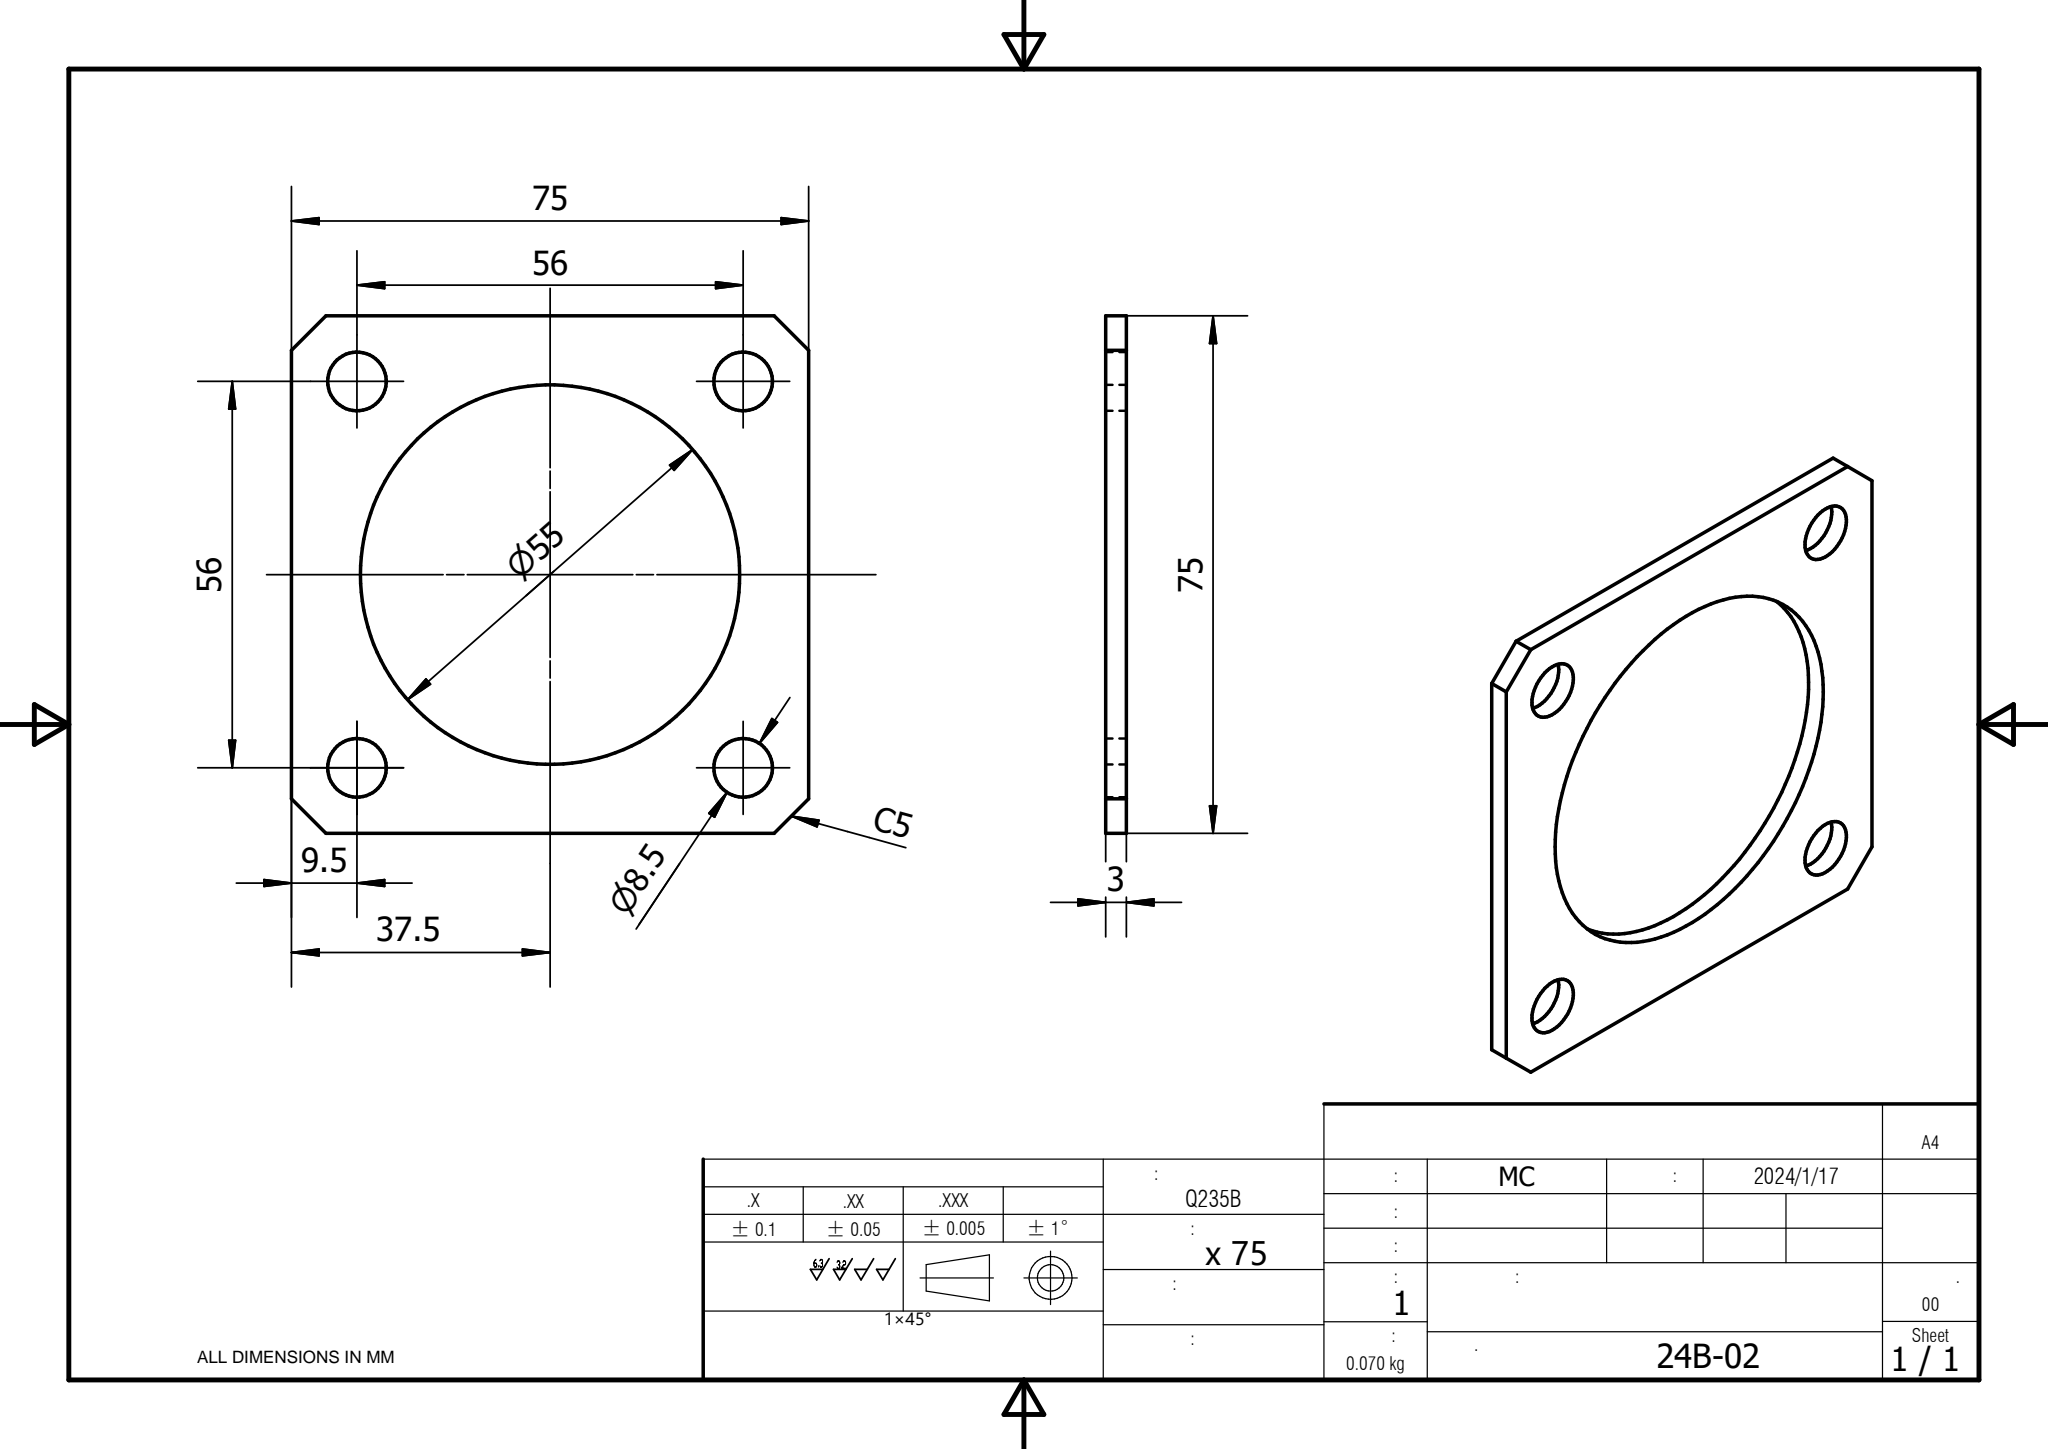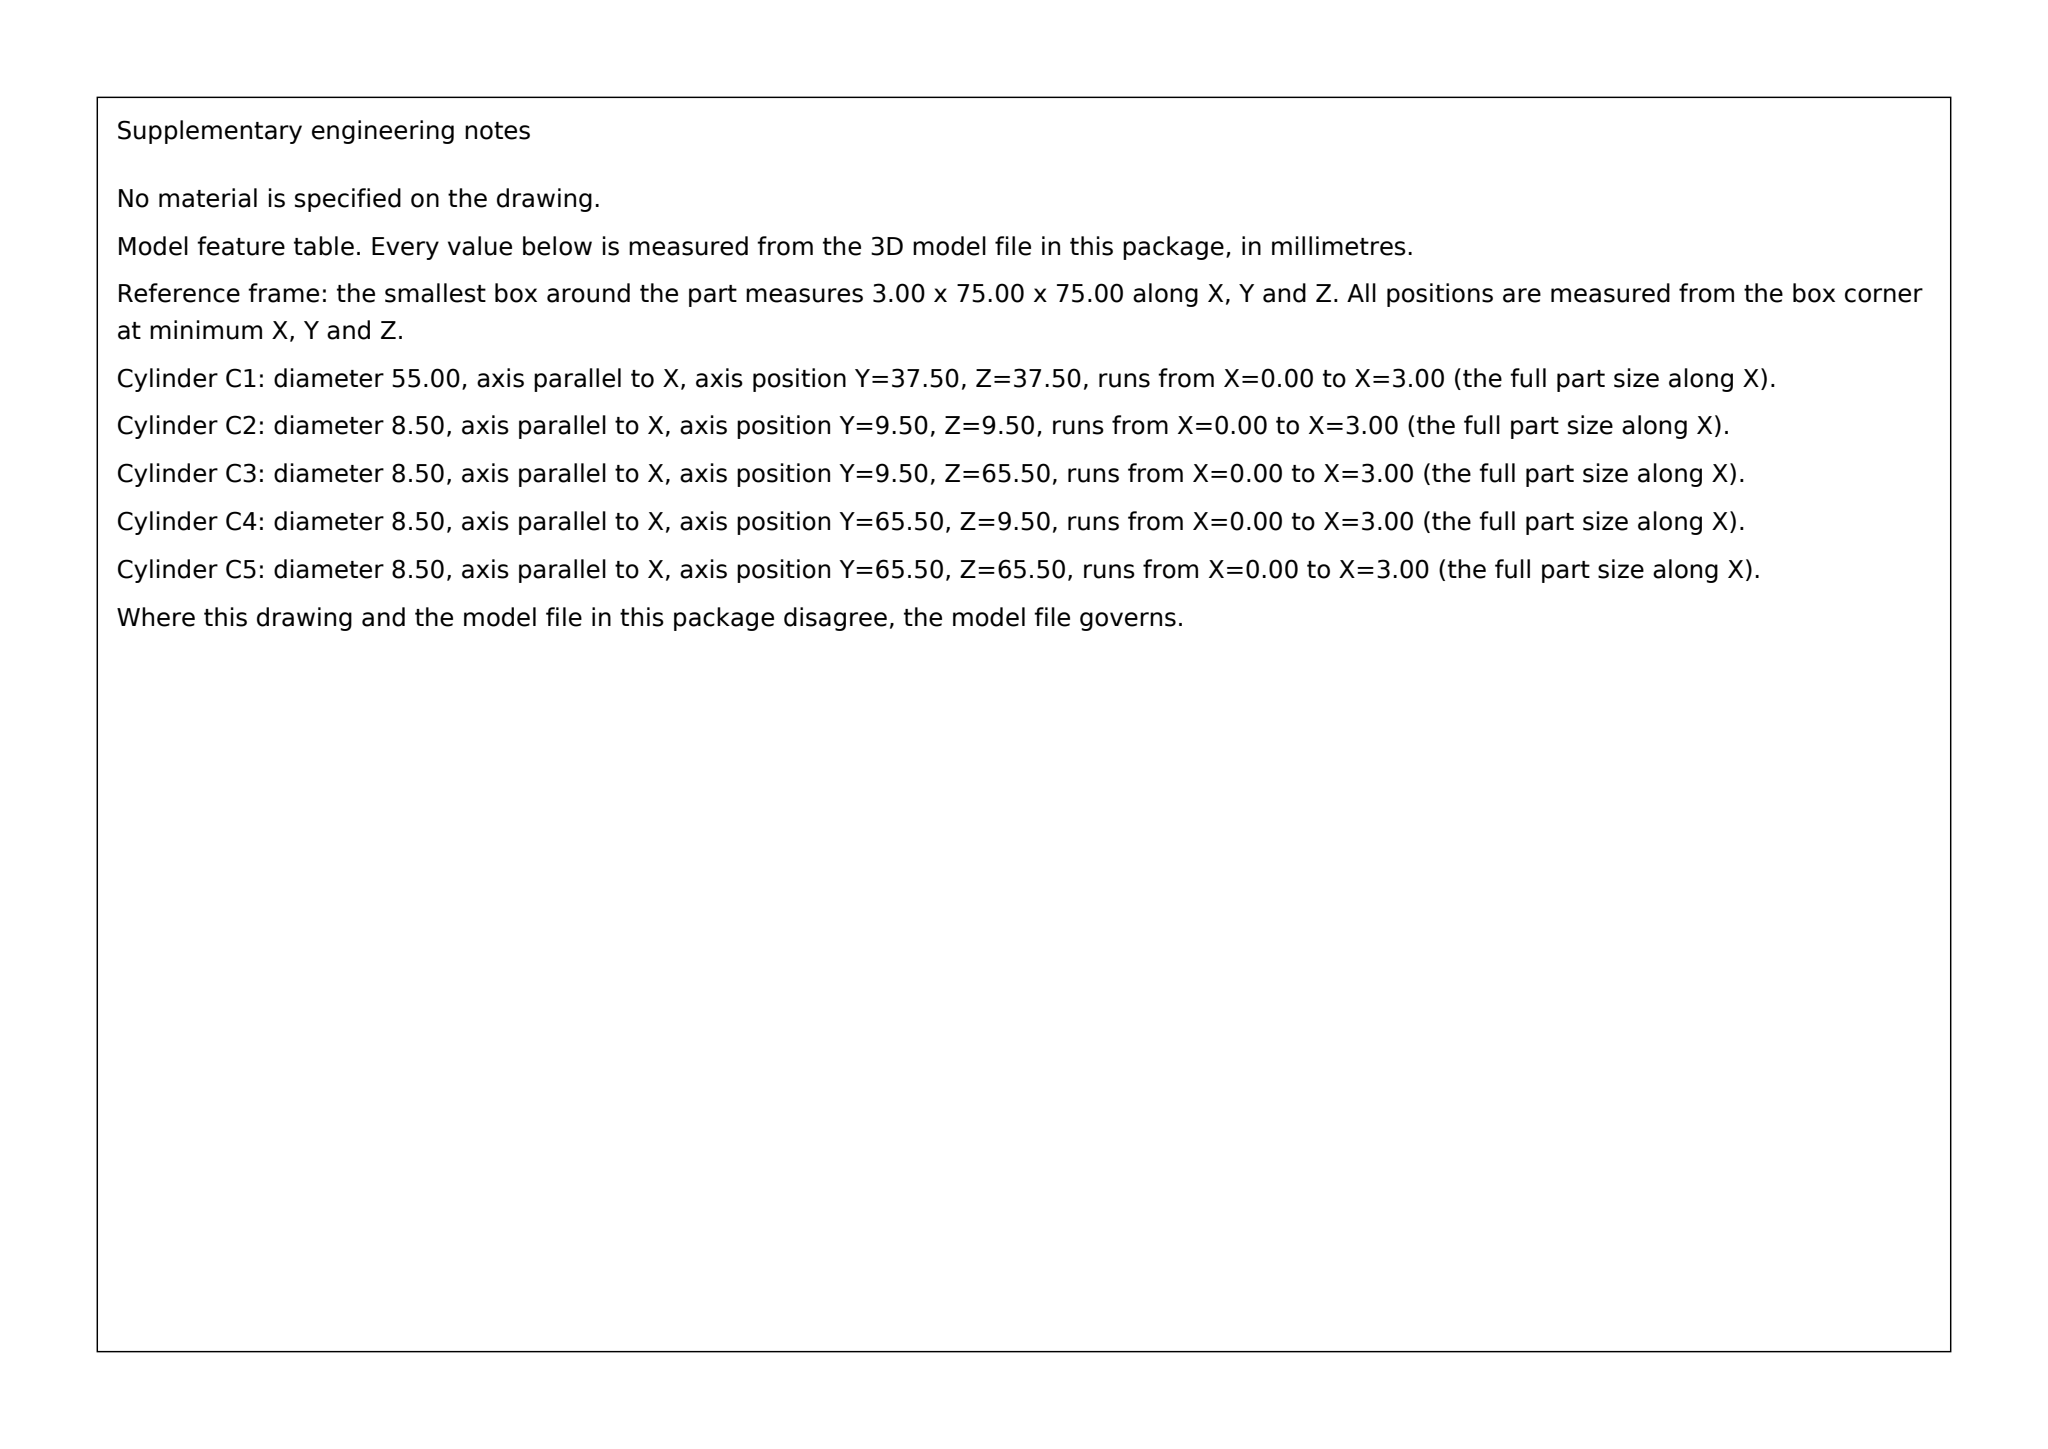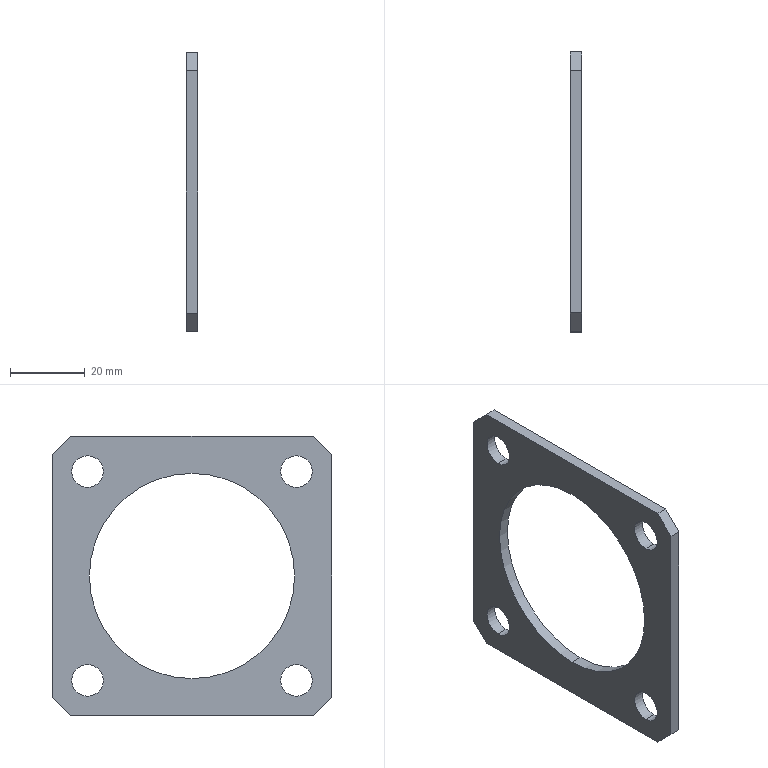Part | SolidWorks | mm | material Q235B | 1 solid | 20 faces | box 3 x 75 x 75 mm | volume 8917 mm3 | cylinder 10 | plane 10 | commonest cylinder face diameters 8.5 x8 55 x2
STEP:
#1=CARTESIAN_POINT('',(3.,0.,-27.5));
#2=VERTEX_POINT('',#1);
#3=CARTESIAN_POINT('',(3.,0.,27.5));
#4=VERTEX_POINT('',#3);
#5=CARTESIAN_POINT('',(3.,0.,0.));
#6=DIRECTION('',(-1.,0.,0.));
#7=DIRECTION('',(0.,0.,1.));
#8=AXIS2_PLACEMENT_3D('',#5,#6,#7);
#9=CIRCLE('',#8,27.5);
#10=EDGE_CURVE('',#2,#4,#9,.T.);
#11=ORIENTED_EDGE('',*,*,#10,.F.);
#12=CARTESIAN_POINT('',(0.,0.,-27.5));
#13=VERTEX_POINT('',#12);
#14=CARTESIAN_POINT('',(3.,0.,-27.5));
#15=DIRECTION('',(-1.,0.,0.));
#16=VECTOR('',#15,1000.);
#17=LINE('',#14,#16);
#18=EDGE_CURVE('',#2,#13,#17,.T.);
#19=ORIENTED_EDGE('',*,*,#18,.T.);
#20=CARTESIAN_POINT('',(0.,0.,27.5));
#21=VERTEX_POINT('',#20);
#22=CARTESIAN_POINT('',(0.,0.,0.));
#23=DIRECTION('',(-1.,0.,0.));
#24=DIRECTION('',(0.,0.,1.));
#25=AXIS2_PLACEMENT_3D('',#22,#23,#24);
#26=CIRCLE('',#25,27.5);
#27=EDGE_CURVE('',#13,#21,#26,.T.);
#28=ORIENTED_EDGE('',*,*,#27,.T.);
#29=CARTESIAN_POINT('',(3.,0.,27.5));
#30=DIRECTION('',(-1.,0.,0.));
#31=VECTOR('',#30,1000.);
#32=LINE('',#29,#31);
#33=EDGE_CURVE('',#4,#21,#32,.T.);
#34=ORIENTED_EDGE('',*,*,#33,.F.);
#35=EDGE_LOOP('',(#11,#19,#28,#34));
#36=FACE_OUTER_BOUND('',#35,.T.);
#37=CARTESIAN_POINT('',(3.,0.,0.));
#38=DIRECTION('',(-1.,0.,0.));
#39=DIRECTION('',(0.,0.,1.));
#40=AXIS2_PLACEMENT_3D('',#37,#38,#39);
#41=CYLINDRICAL_SURFACE('',#40,27.5);
#42=ADVANCED_FACE('',(#36),#41,.F.);
#43=CARTESIAN_POINT('',(0.,-28.,-32.25));
#44=VERTEX_POINT('',#43);
#45=CARTESIAN_POINT('',(0.,-28.,-23.75));
#46=VERTEX_POINT('',#45);
#47=CARTESIAN_POINT('',(0.,-28.,-28.));
#48=DIRECTION('',(-1.,0.,0.));
#49=DIRECTION('',(0.,0.,-1.));
#50=AXIS2_PLACEMENT_3D('',#47,#48,#49);
#51=CIRCLE('',#50,4.25);
#52=EDGE_CURVE('',#44,#46,#51,.T.);
#53=ORIENTED_EDGE('',*,*,#52,.T.);
#54=CARTESIAN_POINT('',(3.,-28.,-23.75));
#55=VERTEX_POINT('',#54);
#56=CARTESIAN_POINT('',(-103.108,-28.,-23.75));
#57=DIRECTION('',(1.,0.,0.));
#58=VECTOR('',#57,1000.);
#59=LINE('',#56,#58);
#60=EDGE_CURVE('',#46,#55,#59,.T.);
#61=ORIENTED_EDGE('',*,*,#60,.T.);
#62=CARTESIAN_POINT('',(3.,-28.,-32.25));
#63=VERTEX_POINT('',#62);
#64=CARTESIAN_POINT('',(3.,-28.,-28.));
#65=DIRECTION('',(-1.,0.,0.));
#66=DIRECTION('',(0.,0.,-1.));
#67=AXIS2_PLACEMENT_3D('',#64,#65,#66);
#68=CIRCLE('',#67,4.25);
#69=EDGE_CURVE('',#63,#55,#68,.T.);
#70=ORIENTED_EDGE('',*,*,#69,.F.);
#71=CARTESIAN_POINT('',(-103.108,-28.,-32.25));
#72=DIRECTION('',(1.,0.,0.));
#73=VECTOR('',#72,1000.);
#74=LINE('',#71,#73);
#75=EDGE_CURVE('',#44,#63,#74,.T.);
#76=ORIENTED_EDGE('',*,*,#75,.F.);
#77=EDGE_LOOP('',(#53,#61,#70,#76));
#78=FACE_OUTER_BOUND('',#77,.T.);
#79=CARTESIAN_POINT('',(-103.108,-28.,-28.));
#80=DIRECTION('',(1.,0.,0.));
#81=DIRECTION('',(0.,0.,-1.));
#82=AXIS2_PLACEMENT_3D('',#79,#80,#81);
#83=CYLINDRICAL_SURFACE('',#82,4.25);
#84=ADVANCED_FACE('',(#78),#83,.F.);
#85=CARTESIAN_POINT('',(0.,28.,-32.25));
#86=VERTEX_POINT('',#85);
#87=CARTESIAN_POINT('',(0.,28.,-23.75));
#88=VERTEX_POINT('',#87);
#89=CARTESIAN_POINT('',(0.,28.,-28.));
#90=DIRECTION('',(-1.,0.,0.));
#91=DIRECTION('',(0.,0.,-1.));
#92=AXIS2_PLACEMENT_3D('',#89,#90,#91);
#93=CIRCLE('',#92,4.25);
#94=EDGE_CURVE('',#86,#88,#93,.T.);
#95=ORIENTED_EDGE('',*,*,#94,.T.);
#96=CARTESIAN_POINT('',(3.,28.,-23.75));
#97=VERTEX_POINT('',#96);
#98=CARTESIAN_POINT('',(-103.108,28.,-23.75));
#99=DIRECTION('',(1.,0.,0.));
#100=VECTOR('',#99,1000.);
#101=LINE('',#98,#100);
#102=EDGE_CURVE('',#88,#97,#101,.T.);
#103=ORIENTED_EDGE('',*,*,#102,.T.);
#104=CARTESIAN_POINT('',(3.,28.,-32.25));
#105=VERTEX_POINT('',#104);
#106=CARTESIAN_POINT('',(3.,28.,-28.));
#107=DIRECTION('',(-1.,0.,0.));
#108=DIRECTION('',(0.,0.,-1.));
#109=AXIS2_PLACEMENT_3D('',#106,#107,#108);
#110=CIRCLE('',#109,4.25);
#111=EDGE_CURVE('',#105,#97,#110,.T.);
#112=ORIENTED_EDGE('',*,*,#111,.F.);
#113=CARTESIAN_POINT('',(-103.108,28.,-32.25));
#114=DIRECTION('',(1.,0.,0.));
#115=VECTOR('',#114,1000.);
#116=LINE('',#113,#115);
#117=EDGE_CURVE('',#86,#105,#116,.T.);
#118=ORIENTED_EDGE('',*,*,#117,.F.);
#119=EDGE_LOOP('',(#95,#103,#112,#118));
#120=FACE_OUTER_BOUND('',#119,.T.);
#121=CARTESIAN_POINT('',(-103.108,28.,-28.));
#122=DIRECTION('',(1.,0.,0.));
#123=DIRECTION('',(0.,0.,-1.));
#124=AXIS2_PLACEMENT_3D('',#121,#122,#123);
#125=CYLINDRICAL_SURFACE('',#124,4.25);
#126=ADVANCED_FACE('',(#120),#125,.F.);
#127=CARTESIAN_POINT('',(0.,28.,23.75));
#128=VERTEX_POINT('',#127);
#129=CARTESIAN_POINT('',(0.,28.,32.25));
#130=VERTEX_POINT('',#129);
#131=CARTESIAN_POINT('',(0.,28.,28.));
#132=DIRECTION('',(-1.,0.,0.));
#133=DIRECTION('',(0.,0.,-1.));
#134=AXIS2_PLACEMENT_3D('',#131,#132,#133);
#135=CIRCLE('',#134,4.25);
#136=EDGE_CURVE('',#128,#130,#135,.T.);
#137=ORIENTED_EDGE('',*,*,#136,.T.);
#138=CARTESIAN_POINT('',(3.,28.,32.25));
#139=VERTEX_POINT('',#138);
#140=CARTESIAN_POINT('',(-103.108,28.,32.25));
#141=DIRECTION('',(1.,0.,0.));
#142=VECTOR('',#141,1000.);
#143=LINE('',#140,#142);
#144=EDGE_CURVE('',#130,#139,#143,.T.);
#145=ORIENTED_EDGE('',*,*,#144,.T.);
#146=CARTESIAN_POINT('',(3.,28.,23.75));
#147=VERTEX_POINT('',#146);
#148=CARTESIAN_POINT('',(3.,28.,28.));
#149=DIRECTION('',(-1.,0.,0.));
#150=DIRECTION('',(0.,0.,-1.));
#151=AXIS2_PLACEMENT_3D('',#148,#149,#150);
#152=CIRCLE('',#151,4.25);
#153=EDGE_CURVE('',#147,#139,#152,.T.);
#154=ORIENTED_EDGE('',*,*,#153,.F.);
#155=CARTESIAN_POINT('',(-103.108,28.,23.75));
#156=DIRECTION('',(1.,0.,0.));
#157=VECTOR('',#156,1000.);
#158=LINE('',#155,#157);
#159=EDGE_CURVE('',#128,#147,#158,.T.);
#160=ORIENTED_EDGE('',*,*,#159,.F.);
#161=EDGE_LOOP('',(#137,#145,#154,#160));
#162=FACE_OUTER_BOUND('',#161,.T.);
#163=CARTESIAN_POINT('',(-103.108,28.,28.));
#164=DIRECTION('',(1.,0.,0.));
#165=DIRECTION('',(0.,0.,-1.));
#166=AXIS2_PLACEMENT_3D('',#163,#164,#165);
#167=CYLINDRICAL_SURFACE('',#166,4.25);
#168=ADVANCED_FACE('',(#162),#167,.F.);
#169=CARTESIAN_POINT('',(0.,-28.,23.75));
#170=VERTEX_POINT('',#169);
#171=CARTESIAN_POINT('',(0.,-28.,32.25));
#172=VERTEX_POINT('',#171);
#173=CARTESIAN_POINT('',(0.,-28.,28.));
#174=DIRECTION('',(-1.,0.,0.));
#175=DIRECTION('',(0.,0.,-1.));
#176=AXIS2_PLACEMENT_3D('',#173,#174,#175);
#177=CIRCLE('',#176,4.25);
#178=EDGE_CURVE('',#170,#172,#177,.T.);
#179=ORIENTED_EDGE('',*,*,#178,.T.);
#180=CARTESIAN_POINT('',(3.,-28.,32.25));
#181=VERTEX_POINT('',#180);
#182=CARTESIAN_POINT('',(-103.108,-28.,32.25));
#183=DIRECTION('',(1.,0.,0.));
#184=VECTOR('',#183,1000.);
#185=LINE('',#182,#184);
#186=EDGE_CURVE('',#172,#181,#185,.T.);
#187=ORIENTED_EDGE('',*,*,#186,.T.);
#188=CARTESIAN_POINT('',(3.,-28.,23.75));
#189=VERTEX_POINT('',#188);
#190=CARTESIAN_POINT('',(3.,-28.,28.));
#191=DIRECTION('',(-1.,0.,0.));
#192=DIRECTION('',(0.,0.,-1.));
#193=AXIS2_PLACEMENT_3D('',#190,#191,#192);
#194=CIRCLE('',#193,4.25);
#195=EDGE_CURVE('',#189,#181,#194,.T.);
#196=ORIENTED_EDGE('',*,*,#195,.F.);
#197=CARTESIAN_POINT('',(-103.108,-28.,23.75));
#198=DIRECTION('',(1.,0.,0.));
#199=VECTOR('',#198,1000.);
#200=LINE('',#197,#199);
#201=EDGE_CURVE('',#170,#189,#200,.T.);
#202=ORIENTED_EDGE('',*,*,#201,.F.);
#203=EDGE_LOOP('',(#179,#187,#196,#202));
#204=FACE_OUTER_BOUND('',#203,.T.);
#205=CARTESIAN_POINT('',(-103.108,-28.,28.));
#206=DIRECTION('',(1.,0.,0.));
#207=DIRECTION('',(0.,0.,-1.));
#208=AXIS2_PLACEMENT_3D('',#205,#206,#207);
#209=CYLINDRICAL_SURFACE('',#208,4.25);
#210=ADVANCED_FACE('',(#204),#209,.F.);
#211=CARTESIAN_POINT('',(0.,0.,0.));
#212=DIRECTION('',(-1.,0.,0.));
#213=DIRECTION('',(0.,0.,1.));
#214=AXIS2_PLACEMENT_3D('',#211,#212,#213);
#215=CIRCLE('',#214,27.5);
#216=EDGE_CURVE('',#21,#13,#215,.T.);
#217=ORIENTED_EDGE('',*,*,#216,.F.);
#218=ORIENTED_EDGE('',*,*,#27,.F.);
#219=EDGE_LOOP('',(#217,#218));
#220=FACE_BOUND('',#219,.T.);
#221=ORIENTED_EDGE('',*,*,#52,.F.);
#222=CARTESIAN_POINT('',(0.,-28.,-28.));
#223=DIRECTION('',(-1.,0.,0.));
#224=DIRECTION('',(0.,0.,-1.));
#225=AXIS2_PLACEMENT_3D('',#222,#223,#224);
#226=CIRCLE('',#225,4.25);
#227=EDGE_CURVE('',#46,#44,#226,.T.);
#228=ORIENTED_EDGE('',*,*,#227,.F.);
#229=EDGE_LOOP('',(#221,#228));
#230=FACE_BOUND('',#229,.T.);
#231=ORIENTED_EDGE('',*,*,#94,.F.);
#232=CARTESIAN_POINT('',(0.,28.,-28.));
#233=DIRECTION('',(-1.,0.,0.));
#234=DIRECTION('',(0.,0.,-1.));
#235=AXIS2_PLACEMENT_3D('',#232,#233,#234);
#236=CIRCLE('',#235,4.25);
#237=EDGE_CURVE('',#88,#86,#236,.T.);
#238=ORIENTED_EDGE('',*,*,#237,.F.);
#239=EDGE_LOOP('',(#231,#238));
#240=FACE_BOUND('',#239,.T.);
#241=ORIENTED_EDGE('',*,*,#136,.F.);
#242=CARTESIAN_POINT('',(0.,28.,28.));
#243=DIRECTION('',(-1.,0.,0.));
#244=DIRECTION('',(0.,0.,-1.));
#245=AXIS2_PLACEMENT_3D('',#242,#243,#244);
#246=CIRCLE('',#245,4.25);
#247=EDGE_CURVE('',#130,#128,#246,.T.);
#248=ORIENTED_EDGE('',*,*,#247,.F.);
#249=EDGE_LOOP('',(#241,#248));
#250=FACE_BOUND('',#249,.T.);
#251=ORIENTED_EDGE('',*,*,#178,.F.);
#252=CARTESIAN_POINT('',(0.,-28.,28.));
#253=DIRECTION('',(-1.,0.,0.));
#254=DIRECTION('',(0.,0.,-1.));
#255=AXIS2_PLACEMENT_3D('',#252,#253,#254);
#256=CIRCLE('',#255,4.25);
#257=EDGE_CURVE('',#172,#170,#256,.T.);
#258=ORIENTED_EDGE('',*,*,#257,.F.);
#259=EDGE_LOOP('',(#251,#258));
#260=FACE_BOUND('',#259,.T.);
#261=CARTESIAN_POINT('',(0.,32.5,37.5));
#262=VERTEX_POINT('',#261);
#263=CARTESIAN_POINT('',(0.,-32.5,37.5));
#264=VERTEX_POINT('',#263);
#265=CARTESIAN_POINT('',(0.,-0.,37.5));
#266=DIRECTION('',(0.,-1.,0.));
#267=VECTOR('',#266,1000.);
#268=LINE('',#265,#267);
#269=EDGE_CURVE('',#262,#264,#268,.T.);
#270=ORIENTED_EDGE('',*,*,#269,.F.);
#271=CARTESIAN_POINT('',(0.,37.5,32.5));
#272=VERTEX_POINT('',#271);
#273=CARTESIAN_POINT('',(0.,37.5,32.5));
#274=DIRECTION('',(0.,-0.7071,0.7071));
#275=VECTOR('',#274,1000.);
#276=LINE('',#273,#275);
#277=EDGE_CURVE('',#272,#262,#276,.T.);
#278=ORIENTED_EDGE('',*,*,#277,.F.);
#279=CARTESIAN_POINT('',(0.,37.5,-32.5));
#280=VERTEX_POINT('',#279);
#281=CARTESIAN_POINT('',(0.,37.5,0.));
#282=DIRECTION('',(0.,0.,1.));
#283=VECTOR('',#282,1000.);
#284=LINE('',#281,#283);
#285=EDGE_CURVE('',#280,#272,#284,.T.);
#286=ORIENTED_EDGE('',*,*,#285,.F.);
#287=CARTESIAN_POINT('',(0.,32.5,-37.5));
#288=VERTEX_POINT('',#287);
#289=CARTESIAN_POINT('',(0.,32.5,-37.5));
#290=DIRECTION('',(0.,0.7071,0.7071));
#291=VECTOR('',#290,1000.);
#292=LINE('',#289,#291);
#293=EDGE_CURVE('',#288,#280,#292,.T.);
#294=ORIENTED_EDGE('',*,*,#293,.F.);
#295=CARTESIAN_POINT('',(0.,-32.5,-37.5));
#296=VERTEX_POINT('',#295);
#297=CARTESIAN_POINT('',(0.,-0.,-37.5));
#298=DIRECTION('',(0.,1.,0.));
#299=VECTOR('',#298,1000.);
#300=LINE('',#297,#299);
#301=EDGE_CURVE('',#296,#288,#300,.T.);
#302=ORIENTED_EDGE('',*,*,#301,.F.);
#303=CARTESIAN_POINT('',(0.,-37.5,-32.5));
#304=VERTEX_POINT('',#303);
#305=CARTESIAN_POINT('',(0.,-37.5,-32.5));
#306=DIRECTION('',(0.,0.7071,-0.7071));
#307=VECTOR('',#306,1000.);
#308=LINE('',#305,#307);
#309=EDGE_CURVE('',#304,#296,#308,.T.);
#310=ORIENTED_EDGE('',*,*,#309,.F.);
#311=CARTESIAN_POINT('',(0.,-37.5,32.5));
#312=VERTEX_POINT('',#311);
#313=CARTESIAN_POINT('',(0.,-37.5,0.));
#314=DIRECTION('',(0.,0.,-1.));
#315=VECTOR('',#314,1000.);
#316=LINE('',#313,#315);
#317=EDGE_CURVE('',#312,#304,#316,.T.);
#318=ORIENTED_EDGE('',*,*,#317,.F.);
#319=CARTESIAN_POINT('',(0.,-32.5,37.5));
#320=DIRECTION('',(0.,-0.7071,-0.7071));
#321=VECTOR('',#320,1000.);
#322=LINE('',#319,#321);
#323=EDGE_CURVE('',#264,#312,#322,.T.);
#324=ORIENTED_EDGE('',*,*,#323,.F.);
#325=EDGE_LOOP('',(#270,#278,#286,#294,#302,#310,#318,#324));
#326=FACE_OUTER_BOUND('',#325,.T.);
#327=CARTESIAN_POINT('',(0.,-0.,0.));
#328=DIRECTION('',(1.,0.,0.));
#329=DIRECTION('',(0.,0.,-1.));
#330=AXIS2_PLACEMENT_3D('',#327,#328,#329);
#331=PLANE('',#330);
#332=ADVANCED_FACE('',(#220,#230,#240,#250,#260,#326),#331,.F.);
#333=ORIENTED_EDGE('',*,*,#18,.F.);
#334=CARTESIAN_POINT('',(3.,0.,0.));
#335=DIRECTION('',(-1.,0.,0.));
#336=DIRECTION('',(0.,0.,1.));
#337=AXIS2_PLACEMENT_3D('',#334,#335,#336);
#338=CIRCLE('',#337,27.5);
#339=EDGE_CURVE('',#4,#2,#338,.T.);
#340=ORIENTED_EDGE('',*,*,#339,.F.);
#341=ORIENTED_EDGE('',*,*,#33,.T.);
#342=ORIENTED_EDGE('',*,*,#216,.T.);
#343=EDGE_LOOP('',(#333,#340,#341,#342));
#344=FACE_OUTER_BOUND('',#343,.T.);
#345=CARTESIAN_POINT('',(3.,0.,0.));
#346=DIRECTION('',(-1.,0.,0.));
#347=DIRECTION('',(0.,0.,1.));
#348=AXIS2_PLACEMENT_3D('',#345,#346,#347);
#349=CYLINDRICAL_SURFACE('',#348,27.5);
#350=ADVANCED_FACE('',(#344),#349,.F.);
#351=ORIENTED_EDGE('',*,*,#60,.F.);
#352=ORIENTED_EDGE('',*,*,#227,.T.);
#353=ORIENTED_EDGE('',*,*,#75,.T.);
#354=CARTESIAN_POINT('',(3.,-28.,-28.));
#355=DIRECTION('',(-1.,0.,0.));
#356=DIRECTION('',(0.,0.,-1.));
#357=AXIS2_PLACEMENT_3D('',#354,#355,#356);
#358=CIRCLE('',#357,4.25);
#359=EDGE_CURVE('',#55,#63,#358,.T.);
#360=ORIENTED_EDGE('',*,*,#359,.F.);
#361=EDGE_LOOP('',(#351,#352,#353,#360));
#362=FACE_OUTER_BOUND('',#361,.T.);
#363=CARTESIAN_POINT('',(-103.108,-28.,-28.));
#364=DIRECTION('',(1.,0.,0.));
#365=DIRECTION('',(0.,0.,-1.));
#366=AXIS2_PLACEMENT_3D('',#363,#364,#365);
#367=CYLINDRICAL_SURFACE('',#366,4.25);
#368=ADVANCED_FACE('',(#362),#367,.F.);
#369=ORIENTED_EDGE('',*,*,#102,.F.);
#370=ORIENTED_EDGE('',*,*,#237,.T.);
#371=ORIENTED_EDGE('',*,*,#117,.T.);
#372=CARTESIAN_POINT('',(3.,28.,-28.));
#373=DIRECTION('',(-1.,0.,0.));
#374=DIRECTION('',(0.,0.,-1.));
#375=AXIS2_PLACEMENT_3D('',#372,#373,#374);
#376=CIRCLE('',#375,4.25);
#377=EDGE_CURVE('',#97,#105,#376,.T.);
#378=ORIENTED_EDGE('',*,*,#377,.F.);
#379=EDGE_LOOP('',(#369,#370,#371,#378));
#380=FACE_OUTER_BOUND('',#379,.T.);
#381=CARTESIAN_POINT('',(-103.108,28.,-28.));
#382=DIRECTION('',(1.,0.,0.));
#383=DIRECTION('',(0.,0.,-1.));
#384=AXIS2_PLACEMENT_3D('',#381,#382,#383);
#385=CYLINDRICAL_SURFACE('',#384,4.25);
#386=ADVANCED_FACE('',(#380),#385,.F.);
#387=ORIENTED_EDGE('',*,*,#144,.F.);
#388=ORIENTED_EDGE('',*,*,#247,.T.);
#389=ORIENTED_EDGE('',*,*,#159,.T.);
#390=CARTESIAN_POINT('',(3.,28.,28.));
#391=DIRECTION('',(-1.,0.,0.));
#392=DIRECTION('',(0.,0.,-1.));
#393=AXIS2_PLACEMENT_3D('',#390,#391,#392);
#394=CIRCLE('',#393,4.25);
#395=EDGE_CURVE('',#139,#147,#394,.T.);
#396=ORIENTED_EDGE('',*,*,#395,.F.);
#397=EDGE_LOOP('',(#387,#388,#389,#396));
#398=FACE_OUTER_BOUND('',#397,.T.);
#399=CARTESIAN_POINT('',(-103.108,28.,28.));
#400=DIRECTION('',(1.,0.,0.));
#401=DIRECTION('',(0.,0.,-1.));
#402=AXIS2_PLACEMENT_3D('',#399,#400,#401);
#403=CYLINDRICAL_SURFACE('',#402,4.25);
#404=ADVANCED_FACE('',(#398),#403,.F.);
#405=ORIENTED_EDGE('',*,*,#186,.F.);
#406=ORIENTED_EDGE('',*,*,#257,.T.);
#407=ORIENTED_EDGE('',*,*,#201,.T.);
#408=CARTESIAN_POINT('',(3.,-28.,28.));
#409=DIRECTION('',(-1.,0.,0.));
#410=DIRECTION('',(0.,0.,-1.));
#411=AXIS2_PLACEMENT_3D('',#408,#409,#410);
#412=CIRCLE('',#411,4.25);
#413=EDGE_CURVE('',#181,#189,#412,.T.);
#414=ORIENTED_EDGE('',*,*,#413,.F.);
#415=EDGE_LOOP('',(#405,#406,#407,#414));
#416=FACE_OUTER_BOUND('',#415,.T.);
#417=CARTESIAN_POINT('',(-103.108,-28.,28.));
#418=DIRECTION('',(1.,0.,0.));
#419=DIRECTION('',(0.,0.,-1.));
#420=AXIS2_PLACEMENT_3D('',#417,#418,#419);
#421=CYLINDRICAL_SURFACE('',#420,4.25);
#422=ADVANCED_FACE('',(#416),#421,.F.);
#423=ORIENTED_EDGE('',*,*,#323,.T.);
#424=CARTESIAN_POINT('',(3.,-37.5,32.5));
#425=VERTEX_POINT('',#424);
#426=CARTESIAN_POINT('',(0.,-37.5,32.5));
#427=DIRECTION('',(1.,0.,0.));
#428=VECTOR('',#427,1000.);
#429=LINE('',#426,#428);
#430=EDGE_CURVE('',#312,#425,#429,.T.);
#431=ORIENTED_EDGE('',*,*,#430,.T.);
#432=CARTESIAN_POINT('',(3.,-32.5,37.5));
#433=VERTEX_POINT('',#432);
#434=CARTESIAN_POINT('',(3.,-35.,35.));
#435=DIRECTION('',(0.,0.7071,0.7071));
#436=VECTOR('',#435,1000.);
#437=LINE('',#434,#436);
#438=EDGE_CURVE('',#425,#433,#437,.T.);
#439=ORIENTED_EDGE('',*,*,#438,.T.);
#440=CARTESIAN_POINT('',(0.,-32.5,37.5));
#441=DIRECTION('',(-1.,0.,0.));
#442=VECTOR('',#441,1000.);
#443=LINE('',#440,#442);
#444=EDGE_CURVE('',#433,#264,#443,.T.);
#445=ORIENTED_EDGE('',*,*,#444,.T.);
#446=EDGE_LOOP('',(#423,#431,#439,#445));
#447=FACE_OUTER_BOUND('',#446,.T.);
#448=CARTESIAN_POINT('',(0.,-35.,35.));
#449=DIRECTION('',(0.,-0.7071,0.7071));
#450=DIRECTION('',(0.,-0.7071,-0.7071));
#451=AXIS2_PLACEMENT_3D('',#448,#449,#450);
#452=PLANE('',#451);
#453=ADVANCED_FACE('',(#447),#452,.T.);
#454=CARTESIAN_POINT('',(3.,32.5,37.5));
#455=VERTEX_POINT('',#454);
#456=CARTESIAN_POINT('',(0.,32.5,37.5));
#457=DIRECTION('',(-1.,0.,0.));
#458=VECTOR('',#457,1000.);
#459=LINE('',#456,#458);
#460=EDGE_CURVE('',#455,#262,#459,.T.);
#461=ORIENTED_EDGE('',*,*,#460,.T.);
#462=ORIENTED_EDGE('',*,*,#269,.T.);
#463=ORIENTED_EDGE('',*,*,#444,.F.);
#464=CARTESIAN_POINT('',(3.,37.5,37.5));
#465=DIRECTION('',(0.,1.,0.));
#466=VECTOR('',#465,1000.);
#467=LINE('',#464,#466);
#468=EDGE_CURVE('',#433,#455,#467,.T.);
#469=ORIENTED_EDGE('',*,*,#468,.T.);
#470=EDGE_LOOP('',(#461,#462,#463,#469));
#471=FACE_OUTER_BOUND('',#470,.T.);
#472=CARTESIAN_POINT('',(0.,37.5,37.5));
#473=DIRECTION('',(0.,-0.,1.));
#474=DIRECTION('',(0.,-1.,-0.));
#475=AXIS2_PLACEMENT_3D('',#472,#473,#474);
#476=PLANE('',#475);
#477=ADVANCED_FACE('',(#471),#476,.T.);
#478=ORIENTED_EDGE('',*,*,#277,.T.);
#479=ORIENTED_EDGE('',*,*,#460,.F.);
#480=CARTESIAN_POINT('',(3.,37.5,32.5));
#481=VERTEX_POINT('',#480);
#482=CARTESIAN_POINT('',(3.,35.,35.));
#483=DIRECTION('',(0.,0.7071,-0.7071));
#484=VECTOR('',#483,1000.);
#485=LINE('',#482,#484);
#486=EDGE_CURVE('',#455,#481,#485,.T.);
#487=ORIENTED_EDGE('',*,*,#486,.T.);
#488=CARTESIAN_POINT('',(0.,37.5,32.5));
#489=DIRECTION('',(-1.,0.,0.));
#490=VECTOR('',#489,1000.);
#491=LINE('',#488,#490);
#492=EDGE_CURVE('',#481,#272,#491,.T.);
#493=ORIENTED_EDGE('',*,*,#492,.T.);
#494=EDGE_LOOP('',(#478,#479,#487,#493));
#495=FACE_OUTER_BOUND('',#494,.T.);
#496=CARTESIAN_POINT('',(0.,35.,35.));
#497=DIRECTION('',(0.,0.7071,0.7071));
#498=DIRECTION('',(0.,-0.7071,0.7071));
#499=AXIS2_PLACEMENT_3D('',#496,#497,#498);
#500=PLANE('',#499);
#501=ADVANCED_FACE('',(#495),#500,.T.);
#502=ORIENTED_EDGE('',*,*,#492,.F.);
#503=CARTESIAN_POINT('',(3.,37.5,-32.5));
#504=VERTEX_POINT('',#503);
#505=CARTESIAN_POINT('',(3.,37.5,-37.5));
#506=DIRECTION('',(0.,0.,-1.));
#507=VECTOR('',#506,1000.);
#508=LINE('',#505,#507);
#509=EDGE_CURVE('',#481,#504,#508,.T.);
#510=ORIENTED_EDGE('',*,*,#509,.T.);
#511=CARTESIAN_POINT('',(0.,37.5,-32.5));
#512=DIRECTION('',(-1.,0.,0.));
#513=VECTOR('',#512,1000.);
#514=LINE('',#511,#513);
#515=EDGE_CURVE('',#504,#280,#514,.T.);
#516=ORIENTED_EDGE('',*,*,#515,.T.);
#517=ORIENTED_EDGE('',*,*,#285,.T.);
#518=EDGE_LOOP('',(#502,#510,#516,#517));
#519=FACE_OUTER_BOUND('',#518,.T.);
#520=CARTESIAN_POINT('',(0.,37.5,-37.5));
#521=DIRECTION('',(0.,1.,0.));
#522=DIRECTION('',(0.,-0.,1.));
#523=AXIS2_PLACEMENT_3D('',#520,#521,#522);
#524=PLANE('',#523);
#525=ADVANCED_FACE('',(#519),#524,.T.);
#526=ORIENTED_EDGE('',*,*,#293,.T.);
#527=ORIENTED_EDGE('',*,*,#515,.F.);
#528=CARTESIAN_POINT('',(3.,32.5,-37.5));
#529=VERTEX_POINT('',#528);
#530=CARTESIAN_POINT('',(3.,35.,-35.));
#531=DIRECTION('',(0.,-0.7071,-0.7071));
#532=VECTOR('',#531,1000.);
#533=LINE('',#530,#532);
#534=EDGE_CURVE('',#504,#529,#533,.T.);
#535=ORIENTED_EDGE('',*,*,#534,.T.);
#536=CARTESIAN_POINT('',(0.,32.5,-37.5));
#537=DIRECTION('',(-1.,0.,0.));
#538=VECTOR('',#537,1000.);
#539=LINE('',#536,#538);
#540=EDGE_CURVE('',#529,#288,#539,.T.);
#541=ORIENTED_EDGE('',*,*,#540,.T.);
#542=EDGE_LOOP('',(#526,#527,#535,#541));
#543=FACE_OUTER_BOUND('',#542,.T.);
#544=CARTESIAN_POINT('',(0.,35.,-35.));
#545=DIRECTION('',(0.,0.7071,-0.7071));
#546=DIRECTION('',(0.,0.7071,0.7071));
#547=AXIS2_PLACEMENT_3D('',#544,#545,#546);
#548=PLANE('',#547);
#549=ADVANCED_FACE('',(#543),#548,.T.);
#550=ORIENTED_EDGE('',*,*,#540,.F.);
#551=CARTESIAN_POINT('',(3.,-32.5,-37.5));
#552=VERTEX_POINT('',#551);
#553=CARTESIAN_POINT('',(3.,-37.5,-37.5));
#554=DIRECTION('',(0.,-1.,0.));
#555=VECTOR('',#554,1000.);
#556=LINE('',#553,#555);
#557=EDGE_CURVE('',#529,#552,#556,.T.);
#558=ORIENTED_EDGE('',*,*,#557,.T.);
#559=CARTESIAN_POINT('',(0.,-32.5,-37.5));
#560=DIRECTION('',(-1.,0.,0.));
#561=VECTOR('',#560,1000.);
#562=LINE('',#559,#561);
#563=EDGE_CURVE('',#552,#296,#562,.T.);
#564=ORIENTED_EDGE('',*,*,#563,.T.);
#565=ORIENTED_EDGE('',*,*,#301,.T.);
#566=EDGE_LOOP('',(#550,#558,#564,#565));
#567=FACE_OUTER_BOUND('',#566,.T.);
#568=CARTESIAN_POINT('',(0.,-37.5,-37.5));
#569=DIRECTION('',(0.,0.,-1.));
#570=DIRECTION('',(-1.,0.,0.));
#571=AXIS2_PLACEMENT_3D('',#568,#569,#570);
#572=PLANE('',#571);
#573=ADVANCED_FACE('',(#567),#572,.T.);
#574=ORIENTED_EDGE('',*,*,#309,.T.);
#575=ORIENTED_EDGE('',*,*,#563,.F.);
#576=CARTESIAN_POINT('',(3.,-37.5,-32.5));
#577=VERTEX_POINT('',#576);
#578=CARTESIAN_POINT('',(3.,-35.,-35.));
#579=DIRECTION('',(0.,-0.7071,0.7071));
#580=VECTOR('',#579,1000.);
#581=LINE('',#578,#580);
#582=EDGE_CURVE('',#552,#577,#581,.T.);
#583=ORIENTED_EDGE('',*,*,#582,.T.);
#584=CARTESIAN_POINT('',(0.,-37.5,-32.5));
#585=DIRECTION('',(-1.,0.,0.));
#586=VECTOR('',#585,1000.);
#587=LINE('',#584,#586);
#588=EDGE_CURVE('',#577,#304,#587,.T.);
#589=ORIENTED_EDGE('',*,*,#588,.T.);
#590=EDGE_LOOP('',(#574,#575,#583,#589));
#591=FACE_OUTER_BOUND('',#590,.T.);
#592=CARTESIAN_POINT('',(0.,-35.,-35.));
#593=DIRECTION('',(0.,-0.7071,-0.7071));
#594=DIRECTION('',(0.,0.7071,-0.7071));
#595=AXIS2_PLACEMENT_3D('',#592,#593,#594);
#596=PLANE('',#595);
#597=ADVANCED_FACE('',(#591),#596,.T.);
#598=ORIENTED_EDGE('',*,*,#588,.F.);
#599=CARTESIAN_POINT('',(3.,-37.5,37.5));
#600=DIRECTION('',(0.,0.,1.));
#601=VECTOR('',#600,1000.);
#602=LINE('',#599,#601);
#603=EDGE_CURVE('',#577,#425,#602,.T.);
#604=ORIENTED_EDGE('',*,*,#603,.T.);
#605=ORIENTED_EDGE('',*,*,#430,.F.);
#606=ORIENTED_EDGE('',*,*,#317,.T.);
#607=EDGE_LOOP('',(#598,#604,#605,#606));
#608=FACE_OUTER_BOUND('',#607,.T.);
#609=CARTESIAN_POINT('',(0.,-37.5,37.5));
#610=DIRECTION('',(0.,-1.,0.));
#611=DIRECTION('',(0.,0.,-1.));
#612=AXIS2_PLACEMENT_3D('',#609,#610,#611);
#613=PLANE('',#612);
#614=ADVANCED_FACE('',(#608),#613,.T.);
#615=ORIENTED_EDGE('',*,*,#339,.T.);
#616=ORIENTED_EDGE('',*,*,#10,.T.);
#617=EDGE_LOOP('',(#615,#616));
#618=FACE_BOUND('',#617,.T.);
#619=ORIENTED_EDGE('',*,*,#69,.T.);
#620=ORIENTED_EDGE('',*,*,#359,.T.);
#621=EDGE_LOOP('',(#619,#620));
#622=FACE_BOUND('',#621,.T.);
#623=ORIENTED_EDGE('',*,*,#111,.T.);
#624=ORIENTED_EDGE('',*,*,#377,.T.);
#625=EDGE_LOOP('',(#623,#624));
#626=FACE_BOUND('',#625,.T.);
#627=ORIENTED_EDGE('',*,*,#153,.T.);
#628=ORIENTED_EDGE('',*,*,#395,.T.);
#629=EDGE_LOOP('',(#627,#628));
#630=FACE_BOUND('',#629,.T.);
#631=ORIENTED_EDGE('',*,*,#195,.T.);
#632=ORIENTED_EDGE('',*,*,#413,.T.);
#633=EDGE_LOOP('',(#631,#632));
#634=FACE_BOUND('',#633,.T.);
#635=ORIENTED_EDGE('',*,*,#486,.F.);
#636=ORIENTED_EDGE('',*,*,#468,.F.);
#637=ORIENTED_EDGE('',*,*,#438,.F.);
#638=ORIENTED_EDGE('',*,*,#603,.F.);
#639=ORIENTED_EDGE('',*,*,#582,.F.);
#640=ORIENTED_EDGE('',*,*,#557,.F.);
#641=ORIENTED_EDGE('',*,*,#534,.F.);
#642=ORIENTED_EDGE('',*,*,#509,.F.);
#643=EDGE_LOOP('',(#635,#636,#637,#638,#639,#640,#641,#642));
#644=FACE_OUTER_BOUND('',#643,.T.);
#645=CARTESIAN_POINT('',(3.,0.,0.));
#646=DIRECTION('',(1.,0.,0.));
#647=DIRECTION('',(0.,0.,-1.));
#648=AXIS2_PLACEMENT_3D('',#645,#646,#647);
#649=PLANE('',#648);
#650=ADVANCED_FACE('',(#618,#622,#626,#630,#634,#644),#649,.T.);
#651=CLOSED_SHELL('',(#42,#84,#126,#168,#210,#332,#350,#368,#386,#404,#422,#453,#477,#501,#525,#549,#573,#597,#614,#650));
#652=MANIFOLD_SOLID_BREP('',#651);
#653=CARTESIAN_POINT('',(0.,0.,0.));
#654=DIRECTION('',(0.,0.,1.));
#655=DIRECTION('',(1.,0.,0.));
#656=AXIS2_PLACEMENT_3D('',#653,#654,#655);
#657=(LENGTH_UNIT()NAMED_UNIT(*)SI_UNIT(.MILLI.,.METRE.));
#658=UNCERTAINTY_MEASURE_WITH_UNIT(LENGTH_MEASURE(0.00001),#657,'','');
#659=(NAMED_UNIT(*)PLANE_ANGLE_UNIT()SI_UNIT($,.RADIAN.));
#660=(NAMED_UNIT(*)SI_UNIT($,.STERADIAN.)SOLID_ANGLE_UNIT());
#661=(GEOMETRIC_REPRESENTATION_CONTEXT(3)GLOBAL_UNCERTAINTY_ASSIGNED_CONTEXT((#658))GLOBAL_UNIT_ASSIGNED_CONTEXT((#657,#659,#660))REPRESENTATION_CONTEXT('',''));
#662=ADVANCED_BREP_SHAPE_REPRESENTATION('',(#652,#656),#661);